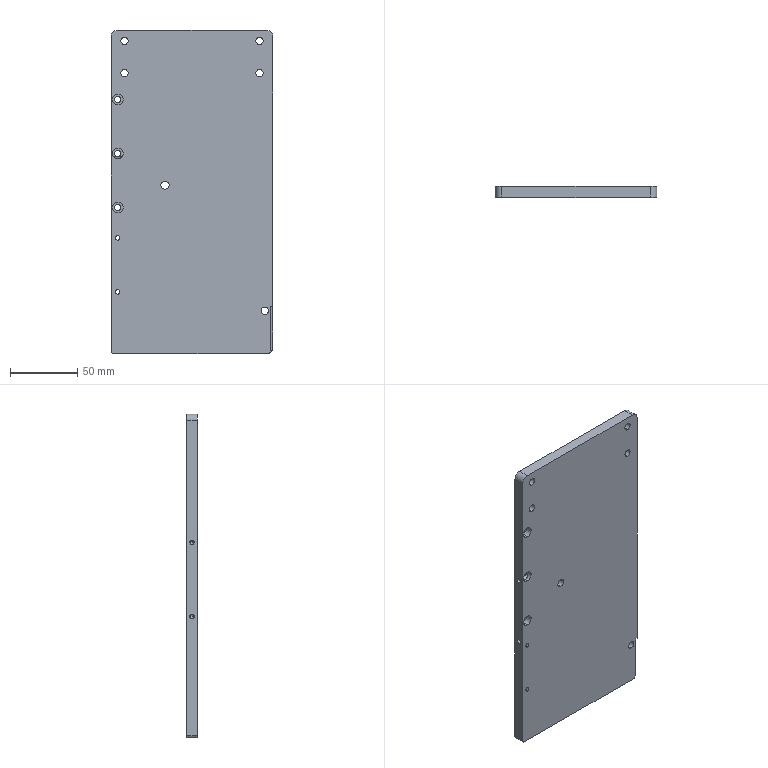Component | SolidWorks | ThirdGenerationFeedingBasePlate-1 | 1 solid | 62 faces | box 120 x 8 x 240 mm | volume 226637 mm3 | cylinder 36 | cone 14 | plane 12 | commonest cylinder face diameters 5.5 x10 3.3 x8 8 x6 4.5 x6 10 x3 6 x2 4 x1
build123d program:
from build123d import *

# Parameters (mm, degrees)
SKETCH1_W                                            = 240
SKETCH1_H                                            = 120
BOSS_EXTRUDE1_DEPTH                                  = 4
M5_HEXAGON_COUNTERSUNK_HEAD_SCREW_TAPERE_D           = 5.5
M5_HEXAGON_COUNTERSUNK_HEAD_SCREW_TAPERE_CSINK_D     = 11.2
M5_HEXAGON_COUNTERSUNK_HEAD_SCREW_TAPERE_CSINK_ANGLE = 90
HOLE_SIZE_ACCORDING_TO_THE_TYPE_OF_HEXAG_D           = 4.5
HOLE_SIZE_ACCORDING_TO_THE_TYPE_OF_HEXAG_CBORE_D     = 8
HOLE_SIZE_ACCORDING_TO_THE_TYPE_OF_HEXAG_CBORE_DEPTH = 4.6
M4_TAPPED_HOLE1_D                                    = 3.3
F_6_0_6_DIAMETER_HOLE1_D                             = 6
F_6_0_6_DIAMETER_HOLE1_DEPTH                         = 10
F_6_0_6_DIAMETER_HOLE1_TIP                           = 1.803
FILLET1_R                                            = 5
M4_TAPPED_HOLE2_D                                    = 3.3
M4_TAPPED_HOLE2_DEPTH                                = 40
M4_TAPPED_HOLE2_TIP                                  = 0.9914
FILLET2_R                                            = 2
SKETCH16_W                                           = 35
SKETCH16_H                                           = 6.5
CUT_EXTRUDE1_DEPTH                                   = 1.5


with BuildPart() as part:
    # Sketch1 → Boss-Extrude1 (new, symmetric)
    with BuildSketch(Plane.XY):
        Rectangle(SKETCH1_W, SKETCH1_H)
    extrude(amount=BOSS_EXTRUDE1_DEPTH, both=True)

    # M5 Hexagon Countersunk Head Screw Tapere (through all)
    with Locations(Plane.XY.offset(4)):
        with Locations((-112, 50), (-112, -50), (-88, -50), (-88, 50), (88, -54)):
            CounterSinkHole(M5_HEXAGON_COUNTERSUNK_HEAD_SCREW_TAPERE_D / 2, M5_HEXAGON_COUNTERSUNK_HEAD_SCREW_TAPERE_CSINK_D / 2, counter_sink_angle=M5_HEXAGON_COUNTERSUNK_HEAD_SCREW_TAPERE_CSINK_ANGLE)

    # Hole Size according to the type of Hexag (through all)
    with Locations(Plane(origin=(0, 0, -4), x_dir=(-1, 0, 0), z_dir=(0, 0, -1))):
        with Locations((-11.5, 55), (28.5, 55), (68.5, 55)):
            CounterBoreHole(HOLE_SIZE_ACCORDING_TO_THE_TYPE_OF_HEXAG_D / 2, HOLE_SIZE_ACCORDING_TO_THE_TYPE_OF_HEXAG_CBORE_D / 2, HOLE_SIZE_ACCORDING_TO_THE_TYPE_OF_HEXAG_CBORE_DEPTH)

    # M4 Tapped Hole1 (through all)
    with Locations(Plane.XY.offset(4)):
        with Locations((34, 55), (74, 55)):
            Hole(M4_TAPPED_HOLE1_D / 2)

    # 6.0 _6_ Diameter Hole1
    with Locations(Plane.XY.offset(4)):
        with Locations((-5, 20)):
            Hole(F_6_0_6_DIAMETER_HOLE1_D / 2, depth=F_6_0_6_DIAMETER_HOLE1_DEPTH)
            with Locations((0, 0, -(F_6_0_6_DIAMETER_HOLE1_DEPTH + F_6_0_6_DIAMETER_HOLE1_TIP / 2))):  # 118° drill point
                Cone(0, F_6_0_6_DIAMETER_HOLE1_D / 2, F_6_0_6_DIAMETER_HOLE1_TIP, mode=Mode.SUBTRACT)

    # Fillet1
    fillet1_edges = [part.edges().sort_by_distance(p)[0] for p in [
        (120, -60, 0),
        (-120, -60, 0),
        (-120, 60, 0),
    ]]
    fillet(fillet1_edges, radius=FILLET1_R)

    # M4 Tapped Hole2
    with Locations(Plane(origin=(-30.52, 60, 0.4504), x_dir=(-1, 0, 0), z_dir=(0, 1, 0))):
        with Locations((-5.52, -0.4504), (-60.52, -0.4504)):
            Hole(M4_TAPPED_HOLE2_D / 2, depth=M4_TAPPED_HOLE2_DEPTH)
            with Locations((0, 0, -(M4_TAPPED_HOLE2_DEPTH + M4_TAPPED_HOLE2_TIP / 2))):  # 118° drill point
                Cone(0, M4_TAPPED_HOLE2_D / 2, M4_TAPPED_HOLE2_TIP, mode=Mode.SUBTRACT)

    # Fillet2
    fillet2_edges = [part.edges().sort_by_distance(p)[0] for p in [
        (120, 60, 0),
    ]]
    fillet(fillet2_edges, radius=FILLET2_R)

    # Sketch16 → Cut-Extrude1 (cut)
    with BuildSketch(Plane.XZ.offset(60)):
        with Locations((102.5, -0.75)):
            Rectangle(SKETCH16_W, SKETCH16_H)
    extrude(amount=-CUT_EXTRUDE1_DEPTH, mode=Mode.SUBTRACT)


solid = part.part

# Placed as in the assembly
solid = solid.moved(Location((-20.027, 37.863, -100), (-90, 0, 90)))